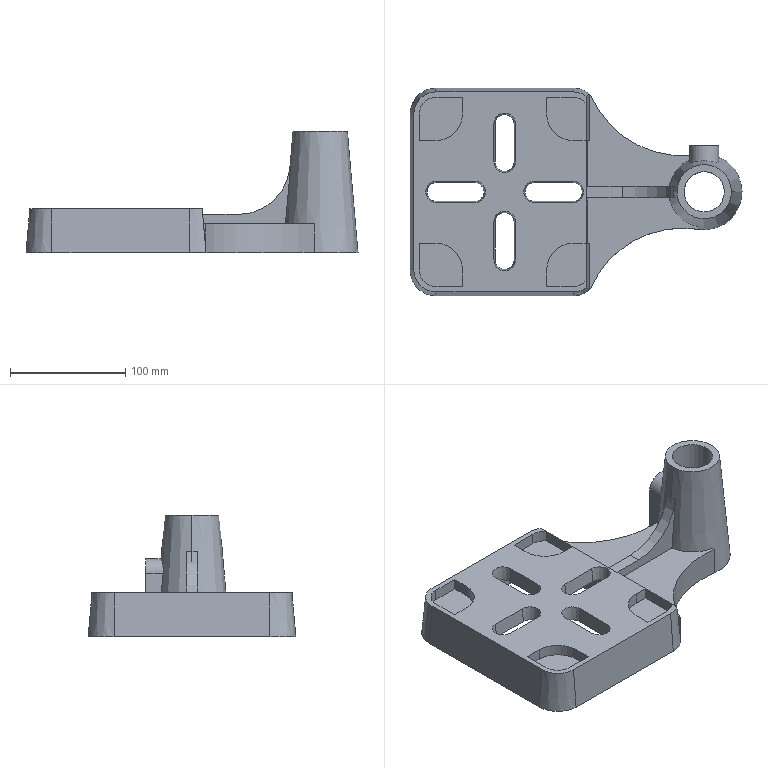Component | SolidWorks | 1New-1 | 3 solids | 102 faces | volume 819478 mm3 | plane 65 | cylinder 20 | cone 17 | commonest cylinder face diameters 46 x8 29 x4 10 x2 35 x2 175 x2 90 x1 25 x1